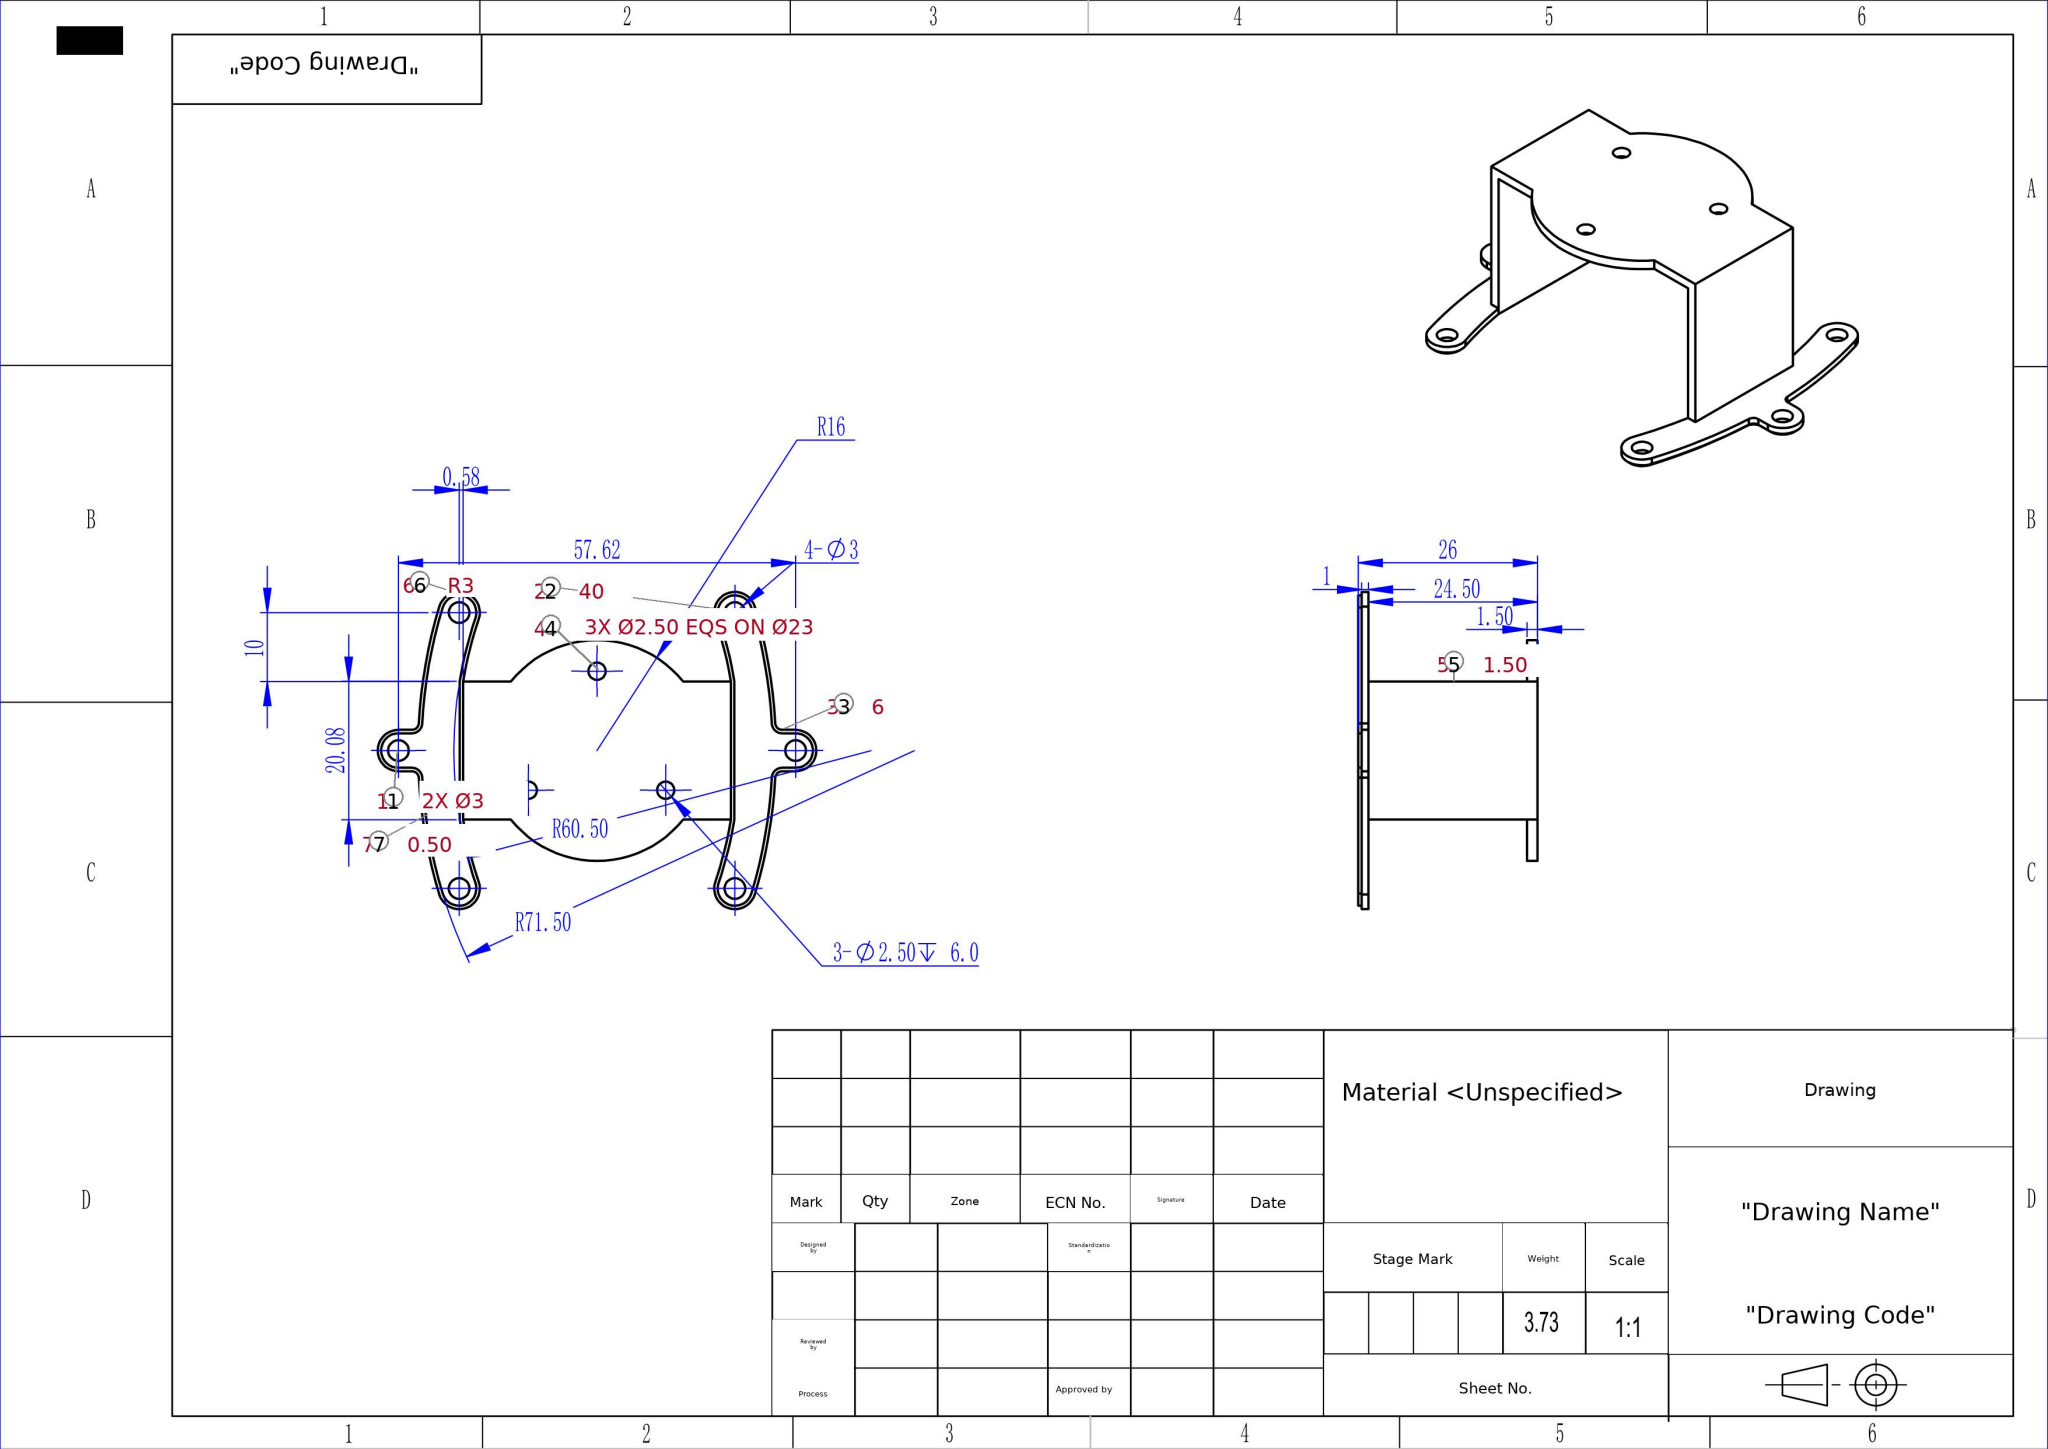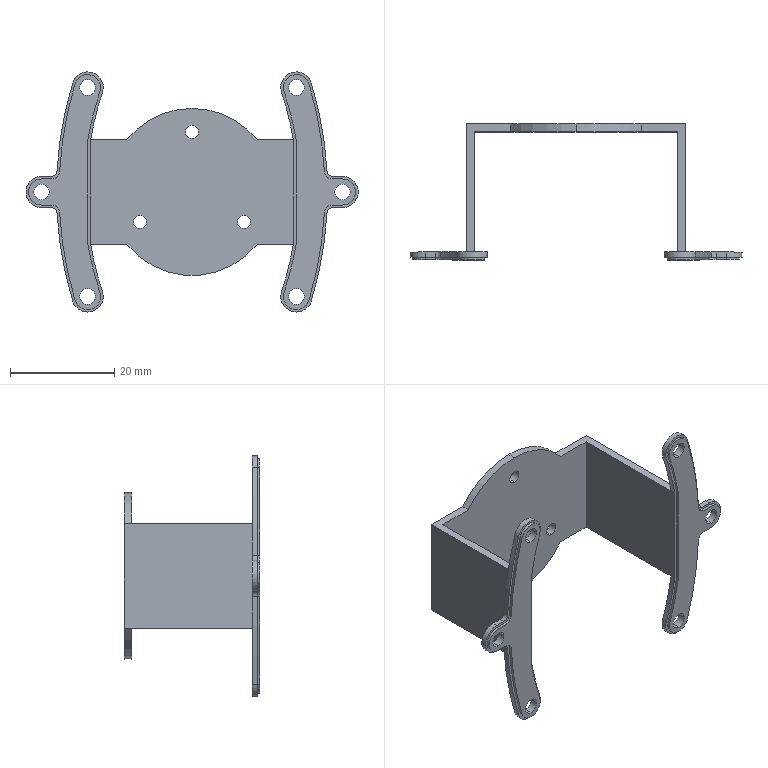Part | SolidWorks | mm | 1 solid | 87 faces | box 63.62 x 26 x 46 mm | volume 3730 mm3 | cylinder 61 | plane 26 | commonest cylinder face diameters 3 x16 5 x8 6 x8 2.5 x6 144 x4 120 x4 2 x4 143 x4